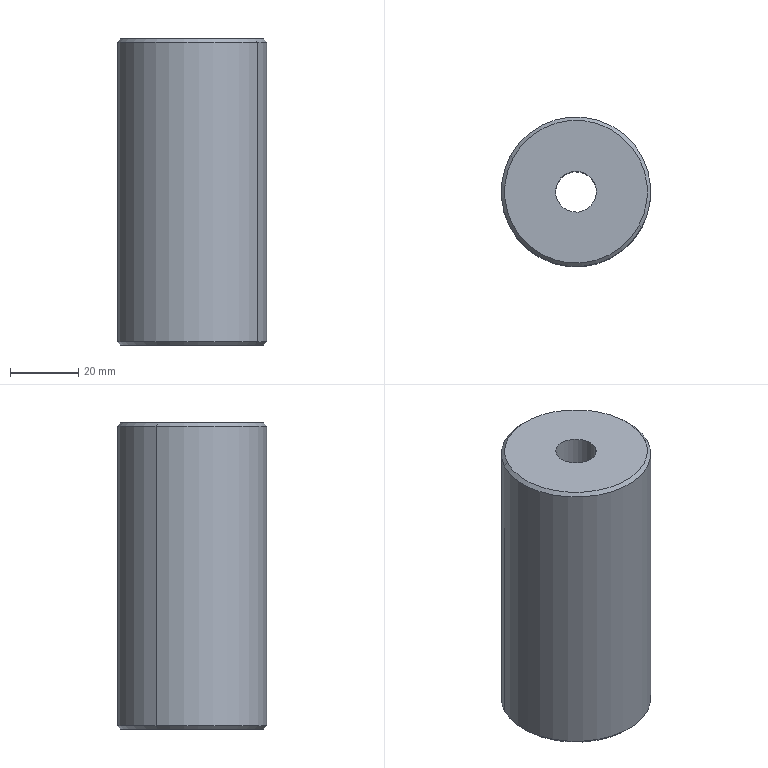Component | SolidWorks | TAR-02-034PaperRollWheel-1 | 1 solid | 10 faces | box 44 x 44 x 90 mm | volume 126533 mm3 | cone 4 | cylinder 4 | plane 2 | commonest cylinder face diameters 12 x2 44 x2
build123d program:
from build123d import *

# Parameters (mm, degrees)
SKETCH1_R           = 22
SKETCH1_R_2         = 6
BOSS_EXTRUDE1_DEPTH = 90
CHAMFER1_SIZE       = 1


with BuildPart() as part:
    # Sketch1 → Boss-Extrude1 (new body)
    with BuildSketch(Plane.XY):
        with Locations(Location((0, 0, 0), (0, 0, 180))):
            Circle(SKETCH1_R)
        with Locations(Location((0, 0, 0), (0, 0, 180))):
            Circle(SKETCH1_R_2, mode=Mode.SUBTRACT)
    extrude(amount=BOSS_EXTRUDE1_DEPTH)

    # Chamfer1
    chamfer1_edges = [part.edges().sort_by_distance(p)[0] for p in [
        (22, 0, 0),
        (22, 0, 90),
    ]]
    chamfer(chamfer1_edges, length=CHAMFER1_SIZE)


solid = part.part

# Placed as in the assembly
solid = solid.moved(Location((14.609, 9.288, -138.439), (0, 0, 0)))
STEP:
#1=CARTESIAN_POINT('',(1.3,-0.03215,-1.907));
#2=VERTEX_POINT('',#1);
#3=CARTESIAN_POINT('',(-0.1496,0.7635,-1.907));
#4=VERTEX_POINT('',#3);
#5=CARTESIAN_POINT('',(0.5752,0.3657,-1.907));
#6=DIRECTION('',(0.,0.,1.));
#7=DIRECTION('',(0.8766,-0.4812,0.));
#8=AXIS2_PLACEMENT_3D('',#5,#6,#7);
#9=CIRCLE('',#8,0.8268);
#10=EDGE_CURVE('',#2,#4,#9,.T.);
#11=ORIENTED_EDGE('',*,*,#10,.F.);
#12=CARTESIAN_POINT('',(1.334,-0.0511,-1.946));
#13=VERTEX_POINT('',#12);
#14=CARTESIAN_POINT('',(1.3,-0.03215,-1.907));
#15=DIRECTION('',(0.6199,-0.3402,-0.7071));
#16=VECTOR('',#15,39.37);
#17=LINE('',#14,#16);
#18=EDGE_CURVE('',#2,#13,#17,.T.);
#19=ORIENTED_EDGE('',*,*,#18,.T.);
#20=CARTESIAN_POINT('',(-0.1841,0.7824,-1.946));
#21=VERTEX_POINT('',#20);
#22=CARTESIAN_POINT('',(0.5752,0.3657,-1.946));
#23=DIRECTION('',(0.,0.,-1.));
#24=DIRECTION('',(0.8766,-0.4812,0.));
#25=AXIS2_PLACEMENT_3D('',#22,#23,#24);
#26=CIRCLE('',#25,0.8661);
#27=EDGE_CURVE('',#21,#13,#26,.T.);
#28=ORIENTED_EDGE('',*,*,#27,.F.);
#29=CARTESIAN_POINT('',(-0.1496,0.7635,-1.907));
#30=DIRECTION('',(-0.6199,0.3402,-0.7071));
#31=VECTOR('',#30,39.37);
#32=LINE('',#29,#31);
#33=EDGE_CURVE('',#4,#21,#32,.T.);
#34=ORIENTED_EDGE('',*,*,#33,.F.);
#35=EDGE_LOOP('',(#11,#19,#28,#34));
#36=FACE_OUTER_BOUND('',#35,.T.);
#37=CARTESIAN_POINT('',(0.5752,0.3657,-1.907));
#38=DIRECTION('',(0.,0.,-1.));
#39=DIRECTION('',(-0.8766,0.4812,0.));
#40=AXIS2_PLACEMENT_3D('',#37,#38,#39);
#41=CONICAL_SURFACE('',#40,0.8268,0.7854);
#42=ADVANCED_FACE('',(#36),#41,.T.);
#43=CARTESIAN_POINT('',(-0.1496,0.7635,-5.45));
#44=VERTEX_POINT('',#43);
#45=CARTESIAN_POINT('',(1.3,-0.03215,-5.45));
#46=VERTEX_POINT('',#45);
#47=CARTESIAN_POINT('',(0.5752,0.3657,-5.45));
#48=DIRECTION('',(0.,0.,-1.));
#49=DIRECTION('',(0.8766,-0.4812,0.));
#50=AXIS2_PLACEMENT_3D('',#47,#48,#49);
#51=CIRCLE('',#50,0.8268);
#52=EDGE_CURVE('',#44,#46,#51,.T.);
#53=ORIENTED_EDGE('',*,*,#52,.F.);
#54=CARTESIAN_POINT('',(-0.1841,0.7824,-5.411));
#55=VERTEX_POINT('',#54);
#56=CARTESIAN_POINT('',(-0.1841,0.7824,-5.411));
#57=DIRECTION('',(-0.6199,0.3402,0.7071));
#58=VECTOR('',#57,39.37);
#59=LINE('',#56,#58);
#60=EDGE_CURVE('',#44,#55,#59,.T.);
#61=ORIENTED_EDGE('',*,*,#60,.T.);
#62=CARTESIAN_POINT('',(1.334,-0.0511,-5.411));
#63=VERTEX_POINT('',#62);
#64=CARTESIAN_POINT('',(0.5752,0.3657,-5.411));
#65=DIRECTION('',(0.,0.,1.));
#66=DIRECTION('',(0.8766,-0.4812,0.));
#67=AXIS2_PLACEMENT_3D('',#64,#65,#66);
#68=CIRCLE('',#67,0.8661);
#69=EDGE_CURVE('',#63,#55,#68,.T.);
#70=ORIENTED_EDGE('',*,*,#69,.F.);
#71=CARTESIAN_POINT('',(1.334,-0.0511,-5.411));
#72=DIRECTION('',(0.6199,-0.3402,0.7071));
#73=VECTOR('',#72,39.37);
#74=LINE('',#71,#73);
#75=EDGE_CURVE('',#46,#63,#74,.T.);
#76=ORIENTED_EDGE('',*,*,#75,.F.);
#77=EDGE_LOOP('',(#53,#61,#70,#76));
#78=FACE_OUTER_BOUND('',#77,.T.);
#79=CARTESIAN_POINT('',(0.5752,0.3657,-5.411));
#80=DIRECTION('',(0.,0.,1.));
#81=DIRECTION('',(0.8766,-0.4812,0.));
#82=AXIS2_PLACEMENT_3D('',#79,#80,#81);
#83=CONICAL_SURFACE('',#82,0.8661,0.7854);
#84=ADVANCED_FACE('',(#78),#83,.T.);
#85=CARTESIAN_POINT('',(0.3681,0.4793,-1.907));
#86=VERTEX_POINT('',#85);
#87=CARTESIAN_POINT('',(0.7822,0.252,-1.907));
#88=VERTEX_POINT('',#87);
#89=CARTESIAN_POINT('',(0.5752,0.3657,-1.907));
#90=DIRECTION('',(0.,0.,1.));
#91=DIRECTION('',(0.8766,-0.4812,0.));
#92=AXIS2_PLACEMENT_3D('',#89,#90,#91);
#93=CIRCLE('',#92,0.2362);
#94=EDGE_CURVE('',#86,#88,#93,.T.);
#95=ORIENTED_EDGE('',*,*,#94,.T.);
#96=CARTESIAN_POINT('',(0.7822,0.252,-5.45));
#97=VERTEX_POINT('',#96);
#98=CARTESIAN_POINT('',(0.7822,0.252,-1.907));
#99=DIRECTION('',(0.,0.,-1.));
#100=VECTOR('',#99,39.37);
#101=LINE('',#98,#100);
#102=EDGE_CURVE('',#88,#97,#101,.T.);
#103=ORIENTED_EDGE('',*,*,#102,.T.);
#104=CARTESIAN_POINT('',(0.3681,0.4793,-5.45));
#105=VERTEX_POINT('',#104);
#106=CARTESIAN_POINT('',(0.5752,0.3657,-5.45));
#107=DIRECTION('',(0.,0.,1.));
#108=DIRECTION('',(0.8766,-0.4812,0.));
#109=AXIS2_PLACEMENT_3D('',#106,#107,#108);
#110=CIRCLE('',#109,0.2362);
#111=EDGE_CURVE('',#105,#97,#110,.T.);
#112=ORIENTED_EDGE('',*,*,#111,.F.);
#113=CARTESIAN_POINT('',(0.3681,0.4793,-1.907));
#114=DIRECTION('',(0.,0.,-1.));
#115=VECTOR('',#114,39.37);
#116=LINE('',#113,#115);
#117=EDGE_CURVE('',#86,#105,#116,.T.);
#118=ORIENTED_EDGE('',*,*,#117,.F.);
#119=EDGE_LOOP('',(#95,#103,#112,#118));
#120=FACE_OUTER_BOUND('',#119,.T.);
#121=CARTESIAN_POINT('',(0.5752,0.3657,-1.907));
#122=DIRECTION('',(0.,0.,-1.));
#123=DIRECTION('',(-0.8766,0.4812,0.));
#124=AXIS2_PLACEMENT_3D('',#121,#122,#123);
#125=CYLINDRICAL_SURFACE('',#124,0.2362);
#126=ADVANCED_FACE('',(#120),#125,.F.);
#127=ORIENTED_EDGE('',*,*,#27,.T.);
#128=CARTESIAN_POINT('',(1.334,-0.0511,-1.907));
#129=DIRECTION('',(0.,0.,-1.));
#130=VECTOR('',#129,39.37);
#131=LINE('',#128,#130);
#132=EDGE_CURVE('',#13,#63,#131,.T.);
#133=ORIENTED_EDGE('',*,*,#132,.T.);
#134=ORIENTED_EDGE('',*,*,#69,.T.);
#135=CARTESIAN_POINT('',(-0.1841,0.7824,-1.907));
#136=DIRECTION('',(0.,0.,-1.));
#137=VECTOR('',#136,39.37);
#138=LINE('',#135,#137);
#139=EDGE_CURVE('',#21,#55,#138,.T.);
#140=ORIENTED_EDGE('',*,*,#139,.F.);
#141=EDGE_LOOP('',(#127,#133,#134,#140));
#142=FACE_OUTER_BOUND('',#141,.T.);
#143=CARTESIAN_POINT('',(0.5752,0.3657,-1.907));
#144=DIRECTION('',(0.,0.,-1.));
#145=DIRECTION('',(-0.8766,0.4812,0.));
#146=AXIS2_PLACEMENT_3D('',#143,#144,#145);
#147=CYLINDRICAL_SURFACE('',#146,0.8661);
#148=ADVANCED_FACE('',(#142),#147,.T.);
#149=CARTESIAN_POINT('',(0.5752,0.3657,-1.907));
#150=DIRECTION('',(0.,0.,1.));
#151=DIRECTION('',(0.8766,-0.4812,0.));
#152=AXIS2_PLACEMENT_3D('',#149,#150,#151);
#153=CIRCLE('',#152,0.8268);
#154=EDGE_CURVE('',#4,#2,#153,.T.);
#155=ORIENTED_EDGE('',*,*,#154,.T.);
#156=ORIENTED_EDGE('',*,*,#10,.T.);
#157=EDGE_LOOP('',(#155,#156));
#158=FACE_OUTER_BOUND('',#157,.T.);
#159=ORIENTED_EDGE('',*,*,#94,.F.);
#160=CARTESIAN_POINT('',(0.5752,0.3657,-1.907));
#161=DIRECTION('',(0.,0.,1.));
#162=DIRECTION('',(0.8766,-0.4812,0.));
#163=AXIS2_PLACEMENT_3D('',#160,#161,#162);
#164=CIRCLE('',#163,0.2362);
#165=EDGE_CURVE('',#88,#86,#164,.T.);
#166=ORIENTED_EDGE('',*,*,#165,.F.);
#167=EDGE_LOOP('',(#159,#166));
#168=FACE_BOUND('',#167,.T.);
#169=CARTESIAN_POINT('',(0.5752,0.3657,-1.907));
#170=DIRECTION('',(0.,0.,1.));
#171=DIRECTION('',(0.8766,-0.4812,0.));
#172=AXIS2_PLACEMENT_3D('',#169,#170,#171);
#173=PLANE('',#172);
#174=ADVANCED_FACE('',(#158,#168),#173,.T.);
#175=CARTESIAN_POINT('',(0.5752,0.3657,-5.45));
#176=DIRECTION('',(0.,0.,-1.));
#177=DIRECTION('',(0.8766,-0.4812,0.));
#178=AXIS2_PLACEMENT_3D('',#175,#176,#177);
#179=CIRCLE('',#178,0.8268);
#180=EDGE_CURVE('',#46,#44,#179,.T.);
#181=ORIENTED_EDGE('',*,*,#180,.T.);
#182=ORIENTED_EDGE('',*,*,#52,.T.);
#183=EDGE_LOOP('',(#181,#182));
#184=FACE_OUTER_BOUND('',#183,.T.);
#185=ORIENTED_EDGE('',*,*,#111,.T.);
#186=CARTESIAN_POINT('',(0.5752,0.3657,-5.45));
#187=DIRECTION('',(0.,0.,1.));
#188=DIRECTION('',(0.8766,-0.4812,0.));
#189=AXIS2_PLACEMENT_3D('',#186,#187,#188);
#190=CIRCLE('',#189,0.2362);
#191=EDGE_CURVE('',#97,#105,#190,.T.);
#192=ORIENTED_EDGE('',*,*,#191,.T.);
#193=EDGE_LOOP('',(#185,#192));
#194=FACE_BOUND('',#193,.T.);
#195=CARTESIAN_POINT('',(0.5752,0.3657,-5.45));
#196=DIRECTION('',(0.,0.,1.));
#197=DIRECTION('',(0.8766,-0.4812,0.));
#198=AXIS2_PLACEMENT_3D('',#195,#196,#197);
#199=PLANE('',#198);
#200=ADVANCED_FACE('',(#184,#194),#199,.F.);
#201=ORIENTED_EDGE('',*,*,#132,.F.);
#202=CARTESIAN_POINT('',(0.5752,0.3657,-1.946));
#203=DIRECTION('',(0.,0.,-1.));
#204=DIRECTION('',(0.8766,-0.4812,0.));
#205=AXIS2_PLACEMENT_3D('',#202,#203,#204);
#206=CIRCLE('',#205,0.8661);
#207=EDGE_CURVE('',#13,#21,#206,.T.);
#208=ORIENTED_EDGE('',*,*,#207,.T.);
#209=ORIENTED_EDGE('',*,*,#139,.T.);
#210=CARTESIAN_POINT('',(0.5752,0.3657,-5.411));
#211=DIRECTION('',(0.,0.,1.));
#212=DIRECTION('',(0.8766,-0.4812,0.));
#213=AXIS2_PLACEMENT_3D('',#210,#211,#212);
#214=CIRCLE('',#213,0.8661);
#215=EDGE_CURVE('',#55,#63,#214,.T.);
#216=ORIENTED_EDGE('',*,*,#215,.T.);
#217=EDGE_LOOP('',(#201,#208,#209,#216));
#218=FACE_OUTER_BOUND('',#217,.T.);
#219=CARTESIAN_POINT('',(0.5752,0.3657,-1.907));
#220=DIRECTION('',(0.,0.,-1.));
#221=DIRECTION('',(-0.8766,0.4812,0.));
#222=AXIS2_PLACEMENT_3D('',#219,#220,#221);
#223=CYLINDRICAL_SURFACE('',#222,0.8661);
#224=ADVANCED_FACE('',(#218),#223,.T.);
#225=ORIENTED_EDGE('',*,*,#102,.F.);
#226=ORIENTED_EDGE('',*,*,#165,.T.);
#227=ORIENTED_EDGE('',*,*,#117,.T.);
#228=ORIENTED_EDGE('',*,*,#191,.F.);
#229=EDGE_LOOP('',(#225,#226,#227,#228));
#230=FACE_OUTER_BOUND('',#229,.T.);
#231=CARTESIAN_POINT('',(0.5752,0.3657,-1.907));
#232=DIRECTION('',(0.,0.,-1.));
#233=DIRECTION('',(-0.8766,0.4812,0.));
#234=AXIS2_PLACEMENT_3D('',#231,#232,#233);
#235=CYLINDRICAL_SURFACE('',#234,0.2362);
#236=ADVANCED_FACE('',(#230),#235,.F.);
#237=ORIENTED_EDGE('',*,*,#60,.F.);
#238=ORIENTED_EDGE('',*,*,#180,.F.);
#239=ORIENTED_EDGE('',*,*,#75,.T.);
#240=ORIENTED_EDGE('',*,*,#215,.F.);
#241=EDGE_LOOP('',(#237,#238,#239,#240));
#242=FACE_OUTER_BOUND('',#241,.T.);
#243=CARTESIAN_POINT('',(0.5752,0.3657,-5.411));
#244=DIRECTION('',(0.,0.,1.));
#245=DIRECTION('',(0.8766,-0.4812,0.));
#246=AXIS2_PLACEMENT_3D('',#243,#244,#245);
#247=CONICAL_SURFACE('',#246,0.8661,0.7854);
#248=ADVANCED_FACE('',(#242),#247,.T.);
#249=ORIENTED_EDGE('',*,*,#18,.F.);
#250=ORIENTED_EDGE('',*,*,#154,.F.);
#251=ORIENTED_EDGE('',*,*,#33,.T.);
#252=ORIENTED_EDGE('',*,*,#207,.F.);
#253=EDGE_LOOP('',(#249,#250,#251,#252));
#254=FACE_OUTER_BOUND('',#253,.T.);
#255=CARTESIAN_POINT('',(0.5752,0.3657,-1.907));
#256=DIRECTION('',(0.,0.,-1.));
#257=DIRECTION('',(-0.8766,0.4812,0.));
#258=AXIS2_PLACEMENT_3D('',#255,#256,#257);
#259=CONICAL_SURFACE('',#258,0.8268,0.7854);
#260=ADVANCED_FACE('',(#254),#259,.T.);
#261=CLOSED_SHELL('',(#42,#84,#126,#148,#174,#200,#224,#236,#248,#260));
#262=MANIFOLD_SOLID_BREP('',#261);
#263=CARTESIAN_POINT('',(0.,0.,0.));
#264=DIRECTION('',(0.,0.,1.));
#265=DIRECTION('',(1.,0.,0.));
#266=AXIS2_PLACEMENT_3D('',#263,#264,#265);
#267=(LENGTH_UNIT()NAMED_UNIT(*)SI_UNIT($,.METRE.));
#268=LENGTH_MEASURE_WITH_UNIT(LENGTH_MEASURE(0.0254),#267);
#269=DIMENSIONAL_EXPONENTS(1.,0.,0.,0.,0.,0.,0.);
#270=(CONVERSION_BASED_UNIT('',#268)LENGTH_UNIT()NAMED_UNIT(#269));
#271=UNCERTAINTY_MEASURE_WITH_UNIT(LENGTH_MEASURE(0.00001),#270,'','');
#272=(NAMED_UNIT(*)PLANE_ANGLE_UNIT()SI_UNIT($,.RADIAN.));
#273=(NAMED_UNIT(*)SI_UNIT($,.STERADIAN.)SOLID_ANGLE_UNIT());
#274=(GEOMETRIC_REPRESENTATION_CONTEXT(3)GLOBAL_UNCERTAINTY_ASSIGNED_CONTEXT((#271))GLOBAL_UNIT_ASSIGNED_CONTEXT((#270,#272,#273))REPRESENTATION_CONTEXT('',''));
#275=ADVANCED_BREP_SHAPE_REPRESENTATION('',(#262,#266),#274);
#276=COLOUR_RGB('',0.7922,0.8196,0.9333);
#277=FILL_AREA_STYLE_COLOUR('',#276);
#278=FILL_AREA_STYLE('',(#277));
#279=SURFACE_STYLE_FILL_AREA(#278);
#280=SURFACE_SIDE_STYLE('',(#279));
#281=SURFACE_STYLE_USAGE(.BOTH.,#280);
#282=PRESENTATION_STYLE_ASSIGNMENT((#281));
#283=STYLED_ITEM('',(#282),#262);
#284=PRESENTATION_LAYER_ASSIGNMENT('','',(#283));
#285=(LENGTH_UNIT()NAMED_UNIT(*)SI_UNIT($,.METRE.));
#286=LENGTH_MEASURE_WITH_UNIT(LENGTH_MEASURE(0.0254),#285);
#287=DIMENSIONAL_EXPONENTS(1.,0.,0.,0.,0.,0.,0.);
#288=(CONVERSION_BASED_UNIT('',#286)LENGTH_UNIT()NAMED_UNIT(#287));
#289=UNCERTAINTY_MEASURE_WITH_UNIT(LENGTH_MEASURE(0.00001),#288,'','');
#290=(NAMED_UNIT(*)PLANE_ANGLE_UNIT()SI_UNIT($,.RADIAN.));
#291=(NAMED_UNIT(*)SI_UNIT($,.STERADIAN.)SOLID_ANGLE_UNIT());
#292=(GEOMETRIC_REPRESENTATION_CONTEXT(3)GLOBAL_UNCERTAINTY_ASSIGNED_CONTEXT((#289))GLOBAL_UNIT_ASSIGNED_CONTEXT((#288,#290,#291))REPRESENTATION_CONTEXT('',''));
#293=MECHANICAL_DESIGN_GEOMETRIC_PRESENTATION_REPRESENTATION('',(#283),#292);